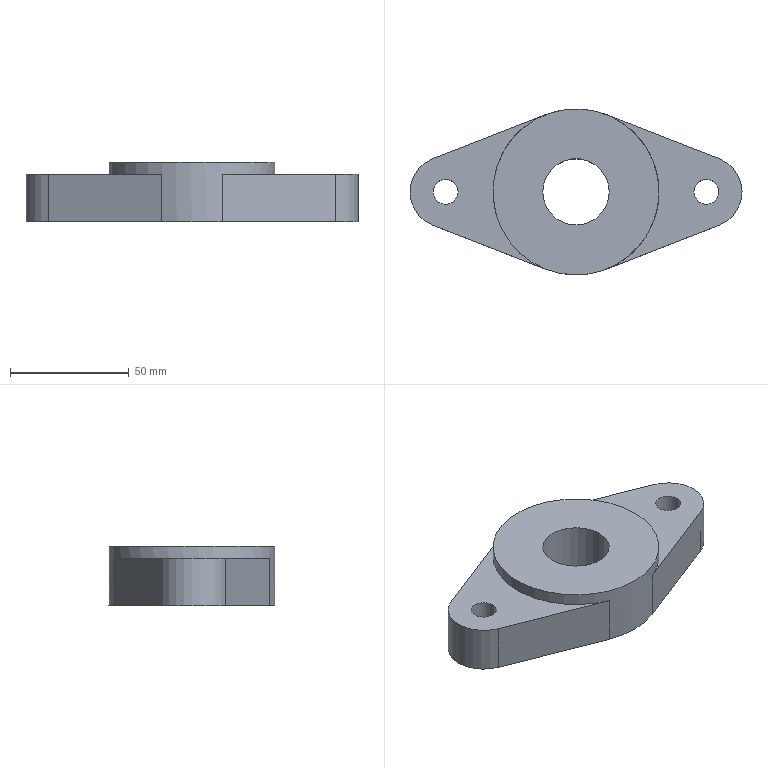Component | NX | FIXED_PLATE | 1 solid | 14 faces | box 140 x 70 x 25 mm | volume 131878 mm3 | plane 8 | cylinder 6 | commonest cylinder face diameters 30 x2 10.5 x2 70 x1 28 x1
STEP:
#1=CARTESIAN_POINT('',(0.,0.,0.));
#2=DIRECTION('',(0.,0.,1.));
#3=DIRECTION('',(1.,0.,0.));
#4=AXIS2_PLACEMENT_3D('',#1,#2,#3);
#5=CARTESIAN_POINT('',(-12.727,-32.604,162.5));
#6=VERTEX_POINT('',#5);
#7=CARTESIAN_POINT('',(-12.727,32.604,162.5));
#8=VERTEX_POINT('',#7);
#9=CARTESIAN_POINT('',(-0.,-0.,162.5));
#10=DIRECTION('',(0.,0.,-1.));
#11=DIRECTION('',(1.,0.,0.));
#12=AXIS2_PLACEMENT_3D('',#9,#10,#11);
#13=CIRCLE('',#12,35.);
#14=CARTESIAN_POINT('',(-55.,-0.,162.5));
#15=DIRECTION('',(0.,0.,1.));
#16=DIRECTION('',(1.,0.,0.));
#17=AXIS2_PLACEMENT_3D('',#14,#15,#16);
#18=PLANE('',#17);
#19=CARTESIAN_POINT('',(90.,0.));
#20=CARTESIAN_POINT('',(90.,-60.622));
#21=CARTESIAN_POINT('',(37.5,-30.311));
#22=CARTESIAN_POINT('',(-15.,-0.));
#23=CARTESIAN_POINT('',(37.5,30.311));
#24=CARTESIAN_POINT('',(90.,60.622));
#25=CARTESIAN_POINT('',(90.,0.));
#26=(BOUNDED_CURVE()B_SPLINE_CURVE(2,(#19,#20,#21,#22,#23,#24,#25),.UNSPECIFIED.,.T.,.F.)B_SPLINE_CURVE_WITH_KNOTS((1,2,2,2,2,1),(-2.094,0.,2.094,4.189,6.283,8.378),.UNSPECIFIED.)CURVE()GEOMETRIC_REPRESENTATION_ITEM()RATIONAL_B_SPLINE_CURVE((1.,0.5,1.,0.5,1.,0.5,1.))REPRESENTATION_ITEM(''));
#27=(GEOMETRIC_REPRESENTATION_CONTEXT(2)PARAMETRIC_REPRESENTATION_CONTEXT()REPRESENTATION_CONTEXT('',''));
#28=DEFINITIONAL_REPRESENTATION('',(#26),#27);
#29=PCURVE('',#18,#28);
#30=CARTESIAN_POINT('',(-0.,-0.,162.5));
#31=DIRECTION('',(0.,0.,-1.));
#32=DIRECTION('',(-1.,0.,0.));
#33=AXIS2_PLACEMENT_3D('',#30,#31,#32);
#34=CYLINDRICAL_SURFACE('',#33,35.);
#35=CARTESIAN_POINT('',(3.142,0.));
#36=DIRECTION('',(1.,0.));
#37=VECTOR('',#36,1.);
#38=LINE('',#35,#37);
#39=(GEOMETRIC_REPRESENTATION_CONTEXT(2)PARAMETRIC_REPRESENTATION_CONTEXT()REPRESENTATION_CONTEXT('',''));
#40=DEFINITIONAL_REPRESENTATION('',(#38),#39);
#41=PCURVE('',#34,#40);
#42=SURFACE_CURVE('',#13,(#29,#41),.PCURVE_S1.);
#43=EDGE_CURVE('',#6,#8,#42,.T.);
#44=ORIENTED_EDGE('',*,*,#43,.T.);
#45=CARTESIAN_POINT('',(-60.455,13.973,162.5));
#46=VERTEX_POINT('',#45);
#47=CARTESIAN_POINT('',(-12.727,32.604,162.5));
#48=DIRECTION('',(-0.9315,-0.3636,0.));
#49=VECTOR('',#48,1.);
#50=LINE('',#47,#49);
#51=CARTESIAN_POINT('',(42.273,32.604));
#52=DIRECTION('',(-0.9315,-0.3636));
#53=VECTOR('',#52,1.);
#54=LINE('',#51,#53);
#55=(GEOMETRIC_REPRESENTATION_CONTEXT(2)PARAMETRIC_REPRESENTATION_CONTEXT()REPRESENTATION_CONTEXT('',''));
#56=DEFINITIONAL_REPRESENTATION('',(#54),#55);
#57=PCURVE('',#18,#56);
#58=CARTESIAN_POINT('',(-12.727,32.604,162.5));
#59=DIRECTION('',(0.3636,-0.9315,0.));
#60=DIRECTION('',(0.9315,0.3636,0.));
#61=AXIS2_PLACEMENT_3D('',#58,#59,#60);
#62=PLANE('',#61);
#63=CARTESIAN_POINT('',(0.,0.));
#64=DIRECTION('',(-1.,0.));
#65=VECTOR('',#64,1.);
#66=LINE('',#63,#65);
#67=(GEOMETRIC_REPRESENTATION_CONTEXT(2)PARAMETRIC_REPRESENTATION_CONTEXT()REPRESENTATION_CONTEXT('',''));
#68=DEFINITIONAL_REPRESENTATION('',(#66),#67);
#69=PCURVE('',#62,#68);
#70=SURFACE_CURVE('',#50,(#57,#69),.PCURVE_S1.);
#71=EDGE_CURVE('',#8,#46,#70,.T.);
#72=ORIENTED_EDGE('',*,*,#71,.T.);
#73=CARTESIAN_POINT('',(-60.455,-13.973,162.5));
#74=VERTEX_POINT('',#73);
#75=CARTESIAN_POINT('',(-55.,-0.,162.5));
#76=DIRECTION('',(0.,0.,1.));
#77=DIRECTION('',(1.,0.,0.));
#78=AXIS2_PLACEMENT_3D('',#75,#76,#77);
#79=CIRCLE('',#78,15.);
#80=CARTESIAN_POINT('',(0.,0.));
#81=DIRECTION('',(1.,0.));
#82=AXIS2_PLACEMENT_2D('',#80,#81);
#83=CIRCLE('',#82,15.);
#84=(GEOMETRIC_REPRESENTATION_CONTEXT(2)PARAMETRIC_REPRESENTATION_CONTEXT()REPRESENTATION_CONTEXT('',''));
#85=DEFINITIONAL_REPRESENTATION('',(#83),#84);
#86=PCURVE('',#18,#85);
#87=CARTESIAN_POINT('',(-55.,-0.,162.5));
#88=DIRECTION('',(0.,0.,-1.));
#89=DIRECTION('',(-1.,0.,0.));
#90=AXIS2_PLACEMENT_3D('',#87,#88,#89);
#91=CYLINDRICAL_SURFACE('',#90,15.);
#92=CARTESIAN_POINT('',(3.142,0.));
#93=DIRECTION('',(-1.,0.));
#94=VECTOR('',#93,1.);
#95=LINE('',#92,#94);
#96=(GEOMETRIC_REPRESENTATION_CONTEXT(2)PARAMETRIC_REPRESENTATION_CONTEXT()REPRESENTATION_CONTEXT('',''));
#97=DEFINITIONAL_REPRESENTATION('',(#95),#96);
#98=PCURVE('',#91,#97);
#99=SURFACE_CURVE('',#79,(#86,#98),.PCURVE_S1.);
#100=EDGE_CURVE('',#46,#74,#99,.T.);
#101=ORIENTED_EDGE('',*,*,#100,.T.);
#102=CARTESIAN_POINT('',(-60.455,-13.973,162.5));
#103=DIRECTION('',(0.9315,-0.3636,0.));
#104=VECTOR('',#103,1.);
#105=LINE('',#102,#104);
#106=CARTESIAN_POINT('',(-5.455,-13.973));
#107=DIRECTION('',(0.9315,-0.3636));
#108=VECTOR('',#107,1.);
#109=LINE('',#106,#108);
#110=(GEOMETRIC_REPRESENTATION_CONTEXT(2)PARAMETRIC_REPRESENTATION_CONTEXT()REPRESENTATION_CONTEXT('',''));
#111=DEFINITIONAL_REPRESENTATION('',(#109),#110);
#112=PCURVE('',#18,#111);
#113=CARTESIAN_POINT('',(-60.455,-13.973,162.5));
#114=DIRECTION('',(0.3636,0.9315,0.));
#115=DIRECTION('',(-0.9315,0.3636,0.));
#116=AXIS2_PLACEMENT_3D('',#113,#114,#115);
#117=PLANE('',#116);
#118=CARTESIAN_POINT('',(0.,0.));
#119=DIRECTION('',(-1.,0.));
#120=VECTOR('',#119,1.);
#121=LINE('',#118,#120);
#122=(GEOMETRIC_REPRESENTATION_CONTEXT(2)PARAMETRIC_REPRESENTATION_CONTEXT()REPRESENTATION_CONTEXT('',''));
#123=DEFINITIONAL_REPRESENTATION('',(#121),#122);
#124=PCURVE('',#117,#123);
#125=SURFACE_CURVE('',#105,(#112,#124),.PCURVE_S1.);
#126=EDGE_CURVE('',#74,#6,#125,.T.);
#127=ORIENTED_EDGE('',*,*,#126,.T.);
#128=EDGE_LOOP('',(#44,#72,#101,#127));
#129=FACE_BOUND('',#128,.T.);
#130=CARTESIAN_POINT('',(-49.75,-0.,162.5));
#131=VERTEX_POINT('',#130);
#132=CARTESIAN_POINT('',(-55.,-0.,162.5));
#133=DIRECTION('',(0.,0.,1.));
#134=DIRECTION('',(1.,0.,0.));
#135=AXIS2_PLACEMENT_3D('',#132,#133,#134);
#136=CIRCLE('',#135,5.25);
#137=CARTESIAN_POINT('',(0.,0.));
#138=DIRECTION('',(1.,0.));
#139=AXIS2_PLACEMENT_2D('',#137,#138);
#140=CIRCLE('',#139,5.25);
#141=(GEOMETRIC_REPRESENTATION_CONTEXT(2)PARAMETRIC_REPRESENTATION_CONTEXT()REPRESENTATION_CONTEXT('',''));
#142=DEFINITIONAL_REPRESENTATION('',(#140),#141);
#143=PCURVE('',#18,#142);
#144=CARTESIAN_POINT('',(-55.,-0.,162.5));
#145=DIRECTION('',(0.,0.,-1.));
#146=DIRECTION('',(-1.,0.,0.));
#147=AXIS2_PLACEMENT_3D('',#144,#145,#146);
#148=CYLINDRICAL_SURFACE('',#147,5.25);
#149=CARTESIAN_POINT('',(9.425,0.));
#150=DIRECTION('',(-1.,0.));
#151=VECTOR('',#150,1.);
#152=LINE('',#149,#151);
#153=(GEOMETRIC_REPRESENTATION_CONTEXT(2)PARAMETRIC_REPRESENTATION_CONTEXT()REPRESENTATION_CONTEXT('',''));
#154=DEFINITIONAL_REPRESENTATION('',(#152),#153);
#155=PCURVE('',#148,#154);
#156=SURFACE_CURVE('',#136,(#143,#155),.PCURVE_S1.);
#157=EDGE_CURVE('',#131,#131,#156,.T.);
#158=ORIENTED_EDGE('',*,*,#157,.F.);
#159=EDGE_LOOP('',(#158));
#160=FACE_BOUND('',#159,.T.);
#161=ADVANCED_FACE('',(#129,#160),#18,.T.);
#162=CARTESIAN_POINT('',(-60.455,13.973,142.5));
#163=VERTEX_POINT('',#162);
#164=CARTESIAN_POINT('',(-60.455,-13.973,142.5));
#165=VERTEX_POINT('',#164);
#166=CARTESIAN_POINT('',(-55.,-0.,142.5));
#167=DIRECTION('',(0.,0.,1.));
#168=DIRECTION('',(1.,0.,0.));
#169=AXIS2_PLACEMENT_3D('',#166,#167,#168);
#170=CIRCLE('',#169,15.);
#171=CARTESIAN_POINT('',(3.142,20.));
#172=DIRECTION('',(-1.,0.));
#173=VECTOR('',#172,1.);
#174=LINE('',#171,#173);
#175=(GEOMETRIC_REPRESENTATION_CONTEXT(2)PARAMETRIC_REPRESENTATION_CONTEXT()REPRESENTATION_CONTEXT('',''));
#176=DEFINITIONAL_REPRESENTATION('',(#174),#175);
#177=PCURVE('',#91,#176);
#178=CARTESIAN_POINT('',(-55.,-0.,142.5));
#179=DIRECTION('',(0.,0.,1.));
#180=DIRECTION('',(1.,0.,0.));
#181=AXIS2_PLACEMENT_3D('',#178,#179,#180);
#182=PLANE('',#181);
#183=CARTESIAN_POINT('',(0.,0.));
#184=DIRECTION('',(1.,0.));
#185=AXIS2_PLACEMENT_2D('',#183,#184);
#186=CIRCLE('',#185,15.);
#187=(GEOMETRIC_REPRESENTATION_CONTEXT(2)PARAMETRIC_REPRESENTATION_CONTEXT()REPRESENTATION_CONTEXT('',''));
#188=DEFINITIONAL_REPRESENTATION('',(#186),#187);
#189=PCURVE('',#182,#188);
#190=SURFACE_CURVE('',#170,(#177,#189),.PCURVE_S1.);
#191=EDGE_CURVE('',#163,#165,#190,.T.);
#192=ORIENTED_EDGE('',*,*,#191,.T.);
#193=CARTESIAN_POINT('',(-60.455,-13.973,162.5));
#194=DIRECTION('',(0.,0.,-1.));
#195=VECTOR('',#194,1.);
#196=LINE('',#193,#195);
#197=CARTESIAN_POINT('',(-1.199,0.));
#198=DIRECTION('',(0.,1.));
#199=VECTOR('',#198,1.);
#200=LINE('',#197,#199);
#201=(GEOMETRIC_REPRESENTATION_CONTEXT(2)PARAMETRIC_REPRESENTATION_CONTEXT()REPRESENTATION_CONTEXT('',''));
#202=DEFINITIONAL_REPRESENTATION('',(#200),#201);
#203=PCURVE('',#91,#202);
#204=CARTESIAN_POINT('',(0.,0.));
#205=DIRECTION('',(0.,-1.));
#206=VECTOR('',#205,1.);
#207=LINE('',#204,#206);
#208=(GEOMETRIC_REPRESENTATION_CONTEXT(2)PARAMETRIC_REPRESENTATION_CONTEXT()REPRESENTATION_CONTEXT('',''));
#209=DEFINITIONAL_REPRESENTATION('',(#207),#208);
#210=PCURVE('',#117,#209);
#211=SURFACE_CURVE('',#196,(#203,#210),.PCURVE_S1.);
#212=EDGE_CURVE('',#74,#165,#211,.T.);
#213=ORIENTED_EDGE('',*,*,#212,.F.);
#214=ORIENTED_EDGE('',*,*,#100,.F.);
#215=CARTESIAN_POINT('',(-60.455,13.973,162.5));
#216=DIRECTION('',(0.,0.,-1.));
#217=VECTOR('',#216,1.);
#218=LINE('',#215,#217);
#219=CARTESIAN_POINT('',(1.199,0.));
#220=DIRECTION('',(0.,1.));
#221=VECTOR('',#220,1.);
#222=LINE('',#219,#221);
#223=(GEOMETRIC_REPRESENTATION_CONTEXT(2)PARAMETRIC_REPRESENTATION_CONTEXT()REPRESENTATION_CONTEXT('',''));
#224=DEFINITIONAL_REPRESENTATION('',(#222),#223);
#225=PCURVE('',#91,#224);
#226=CARTESIAN_POINT('',(-51.235,0.));
#227=DIRECTION('',(0.,-1.));
#228=VECTOR('',#227,1.);
#229=LINE('',#226,#228);
#230=(GEOMETRIC_REPRESENTATION_CONTEXT(2)PARAMETRIC_REPRESENTATION_CONTEXT()REPRESENTATION_CONTEXT('',''));
#231=DEFINITIONAL_REPRESENTATION('',(#229),#230);
#232=PCURVE('',#62,#231);
#233=SURFACE_CURVE('',#218,(#225,#232),.PCURVE_S1.);
#234=EDGE_CURVE('',#46,#163,#233,.T.);
#235=ORIENTED_EDGE('',*,*,#234,.T.);
#236=EDGE_LOOP('',(#192,#213,#214,#235));
#237=FACE_BOUND('',#236,.T.);
#238=ADVANCED_FACE('',(#237),#91,.T.);
#239=CARTESIAN_POINT('',(-12.727,-32.604,142.5));
#240=VERTEX_POINT('',#239);
#241=CARTESIAN_POINT('',(-60.455,-13.973,142.5));
#242=DIRECTION('',(0.9315,-0.3636,0.));
#243=VECTOR('',#242,1.);
#244=LINE('',#241,#243);
#245=CARTESIAN_POINT('',(0.,-20.));
#246=DIRECTION('',(-1.,0.));
#247=VECTOR('',#246,1.);
#248=LINE('',#245,#247);
#249=(GEOMETRIC_REPRESENTATION_CONTEXT(2)PARAMETRIC_REPRESENTATION_CONTEXT()REPRESENTATION_CONTEXT('',''));
#250=DEFINITIONAL_REPRESENTATION('',(#248),#249);
#251=PCURVE('',#117,#250);
#252=CARTESIAN_POINT('',(-5.455,-13.973));
#253=DIRECTION('',(0.9315,-0.3636));
#254=VECTOR('',#253,1.);
#255=LINE('',#252,#254);
#256=(GEOMETRIC_REPRESENTATION_CONTEXT(2)PARAMETRIC_REPRESENTATION_CONTEXT()REPRESENTATION_CONTEXT('',''));
#257=DEFINITIONAL_REPRESENTATION('',(#255),#256);
#258=PCURVE('',#182,#257);
#259=SURFACE_CURVE('',#244,(#251,#258),.PCURVE_S1.);
#260=EDGE_CURVE('',#165,#240,#259,.T.);
#261=ORIENTED_EDGE('',*,*,#260,.T.);
#262=CARTESIAN_POINT('',(-12.727,-32.604,162.5));
#263=DIRECTION('',(0.,0.,-1.));
#264=VECTOR('',#263,1.);
#265=LINE('',#262,#264);
#266=CARTESIAN_POINT('',(-51.235,0.));
#267=DIRECTION('',(0.,-1.));
#268=VECTOR('',#267,1.);
#269=LINE('',#266,#268);
#270=(GEOMETRIC_REPRESENTATION_CONTEXT(2)PARAMETRIC_REPRESENTATION_CONTEXT()REPRESENTATION_CONTEXT('',''));
#271=DEFINITIONAL_REPRESENTATION('',(#269),#270);
#272=PCURVE('',#117,#271);
#273=CARTESIAN_POINT('',(11.368,0.));
#274=DIRECTION('',(0.,1.));
#275=VECTOR('',#274,1.);
#276=LINE('',#273,#275);
#277=(GEOMETRIC_REPRESENTATION_CONTEXT(2)PARAMETRIC_REPRESENTATION_CONTEXT()REPRESENTATION_CONTEXT('',''));
#278=DEFINITIONAL_REPRESENTATION('',(#276),#277);
#279=PCURVE('',#34,#278);
#280=SURFACE_CURVE('',#265,(#272,#279),.PCURVE_S1.);
#281=EDGE_CURVE('',#6,#240,#280,.T.);
#282=ORIENTED_EDGE('',*,*,#281,.F.);
#283=ORIENTED_EDGE('',*,*,#126,.F.);
#284=ORIENTED_EDGE('',*,*,#212,.T.);
#285=EDGE_LOOP('',(#261,#282,#283,#284));
#286=FACE_BOUND('',#285,.T.);
#287=ADVANCED_FACE('',(#286),#117,.F.);
#288=CARTESIAN_POINT('',(12.727,-32.604,142.5));
#289=VERTEX_POINT('',#288);
#290=CARTESIAN_POINT('',(60.455,-13.973,142.5));
#291=VERTEX_POINT('',#290);
#292=CARTESIAN_POINT('',(12.727,-32.604,142.5));
#293=DIRECTION('',(0.9315,0.3636,0.));
#294=VECTOR('',#293,1.);
#295=LINE('',#292,#294);
#296=CARTESIAN_POINT('',(12.727,-32.604,162.5));
#297=DIRECTION('',(-0.3636,0.9315,0.));
#298=DIRECTION('',(-0.9315,-0.3636,0.));
#299=AXIS2_PLACEMENT_3D('',#296,#297,#298);
#300=PLANE('',#299);
#301=CARTESIAN_POINT('',(0.,-20.));
#302=DIRECTION('',(-1.,0.));
#303=VECTOR('',#302,1.);
#304=LINE('',#301,#303);
#305=(GEOMETRIC_REPRESENTATION_CONTEXT(2)PARAMETRIC_REPRESENTATION_CONTEXT()REPRESENTATION_CONTEXT('',''));
#306=DEFINITIONAL_REPRESENTATION('',(#304),#305);
#307=PCURVE('',#300,#306);
#308=CARTESIAN_POINT('',(67.727,-32.604));
#309=DIRECTION('',(0.9315,0.3636));
#310=VECTOR('',#309,1.);
#311=LINE('',#308,#310);
#312=(GEOMETRIC_REPRESENTATION_CONTEXT(2)PARAMETRIC_REPRESENTATION_CONTEXT()REPRESENTATION_CONTEXT('',''));
#313=DEFINITIONAL_REPRESENTATION('',(#311),#312);
#314=PCURVE('',#182,#313);
#315=SURFACE_CURVE('',#295,(#307,#314),.PCURVE_S1.);
#316=EDGE_CURVE('',#289,#291,#315,.T.);
#317=ORIENTED_EDGE('',*,*,#316,.T.);
#318=CARTESIAN_POINT('',(60.455,-13.973,162.5));
#319=VERTEX_POINT('',#318);
#320=CARTESIAN_POINT('',(60.455,-13.973,162.5));
#321=DIRECTION('',(0.,0.,-1.));
#322=VECTOR('',#321,1.);
#323=LINE('',#320,#322);
#324=CARTESIAN_POINT('',(-51.235,0.));
#325=DIRECTION('',(0.,-1.));
#326=VECTOR('',#325,1.);
#327=LINE('',#324,#326);
#328=(GEOMETRIC_REPRESENTATION_CONTEXT(2)PARAMETRIC_REPRESENTATION_CONTEXT()REPRESENTATION_CONTEXT('',''));
#329=DEFINITIONAL_REPRESENTATION('',(#327),#328);
#330=PCURVE('',#300,#329);
#331=CARTESIAN_POINT('',(55.,-0.,162.5));
#332=DIRECTION('',(0.,0.,-1.));
#333=DIRECTION('',(-1.,0.,0.));
#334=AXIS2_PLACEMENT_3D('',#331,#332,#333);
#335=CYLINDRICAL_SURFACE('',#334,15.);
#336=CARTESIAN_POINT('',(4.34,0.));
#337=DIRECTION('',(0.,1.));
#338=VECTOR('',#337,1.);
#339=LINE('',#336,#338);
#340=(GEOMETRIC_REPRESENTATION_CONTEXT(2)PARAMETRIC_REPRESENTATION_CONTEXT()REPRESENTATION_CONTEXT('',''));
#341=DEFINITIONAL_REPRESENTATION('',(#339),#340);
#342=PCURVE('',#335,#341);
#343=SURFACE_CURVE('',#323,(#330,#342),.PCURVE_S1.);
#344=EDGE_CURVE('',#319,#291,#343,.T.);
#345=ORIENTED_EDGE('',*,*,#344,.F.);
#346=CARTESIAN_POINT('',(12.727,-32.604,162.5));
#347=VERTEX_POINT('',#346);
#348=CARTESIAN_POINT('',(12.727,-32.604,162.5));
#349=DIRECTION('',(0.9315,0.3636,0.));
#350=VECTOR('',#349,1.);
#351=LINE('',#348,#350);
#352=CARTESIAN_POINT('',(0.,0.));
#353=DIRECTION('',(-1.,0.));
#354=VECTOR('',#353,1.);
#355=LINE('',#352,#354);
#356=(GEOMETRIC_REPRESENTATION_CONTEXT(2)PARAMETRIC_REPRESENTATION_CONTEXT()REPRESENTATION_CONTEXT('',''));
#357=DEFINITIONAL_REPRESENTATION('',(#355),#356);
#358=PCURVE('',#300,#357);
#359=CARTESIAN_POINT('',(-55.,-0.,162.5));
#360=DIRECTION('',(0.,0.,1.));
#361=DIRECTION('',(1.,0.,0.));
#362=AXIS2_PLACEMENT_3D('',#359,#360,#361);
#363=PLANE('',#362);
#364=CARTESIAN_POINT('',(67.727,-32.604));
#365=DIRECTION('',(0.9315,0.3636));
#366=VECTOR('',#365,1.);
#367=LINE('',#364,#366);
#368=(GEOMETRIC_REPRESENTATION_CONTEXT(2)PARAMETRIC_REPRESENTATION_CONTEXT()REPRESENTATION_CONTEXT('',''));
#369=DEFINITIONAL_REPRESENTATION('',(#367),#368);
#370=PCURVE('',#363,#369);
#371=SURFACE_CURVE('',#351,(#358,#370),.PCURVE_S1.);
#372=EDGE_CURVE('',#347,#319,#371,.T.);
#373=ORIENTED_EDGE('',*,*,#372,.F.);
#374=CARTESIAN_POINT('',(12.727,-32.604,162.5));
#375=DIRECTION('',(0.,0.,-1.));
#376=VECTOR('',#375,1.);
#377=LINE('',#374,#376);
#378=CARTESIAN_POINT('',(0.,0.));
#379=DIRECTION('',(0.,-1.));
#380=VECTOR('',#379,1.);
#381=LINE('',#378,#380);
#382=(GEOMETRIC_REPRESENTATION_CONTEXT(2)PARAMETRIC_REPRESENTATION_CONTEXT()REPRESENTATION_CONTEXT('',''));
#383=DEFINITIONAL_REPRESENTATION('',(#381),#382);
#384=PCURVE('',#300,#383);
#385=CARTESIAN_POINT('',(10.623,0.));
#386=DIRECTION('',(0.,1.));
#387=VECTOR('',#386,1.);
#388=LINE('',#385,#387);
#389=(GEOMETRIC_REPRESENTATION_CONTEXT(2)PARAMETRIC_REPRESENTATION_CONTEXT()REPRESENTATION_CONTEXT('',''));
#390=DEFINITIONAL_REPRESENTATION('',(#388),#389);
#391=PCURVE('',#34,#390);
#392=SURFACE_CURVE('',#377,(#384,#391),.PCURVE_S1.);
#393=EDGE_CURVE('',#347,#289,#392,.T.);
#394=ORIENTED_EDGE('',*,*,#393,.T.);
#395=EDGE_LOOP('',(#317,#345,#373,#394));
#396=FACE_BOUND('',#395,.T.);
#397=ADVANCED_FACE('',(#396),#300,.F.);
#398=CARTESIAN_POINT('',(60.455,13.973,142.5));
#399=VERTEX_POINT('',#398);
#400=CARTESIAN_POINT('',(55.,-0.,142.5));
#401=DIRECTION('',(0.,0.,1.));
#402=DIRECTION('',(-1.,0.,0.));
#403=AXIS2_PLACEMENT_3D('',#400,#401,#402);
#404=CIRCLE('',#403,15.);
#405=CARTESIAN_POINT('',(6.283,20.));
#406=DIRECTION('',(-1.,0.));
#407=VECTOR('',#406,1.);
#408=LINE('',#405,#407);
#409=(GEOMETRIC_REPRESENTATION_CONTEXT(2)PARAMETRIC_REPRESENTATION_CONTEXT()REPRESENTATION_CONTEXT('',''));
#410=DEFINITIONAL_REPRESENTATION('',(#408),#409);
#411=PCURVE('',#335,#410);
#412=CARTESIAN_POINT('',(110.,0.));
#413=DIRECTION('',(-1.,0.));
#414=AXIS2_PLACEMENT_2D('',#412,#413);
#415=CIRCLE('',#414,15.);
#416=(GEOMETRIC_REPRESENTATION_CONTEXT(2)PARAMETRIC_REPRESENTATION_CONTEXT()REPRESENTATION_CONTEXT('',''));
#417=DEFINITIONAL_REPRESENTATION('',(#415),#416);
#418=PCURVE('',#182,#417);
#419=SURFACE_CURVE('',#404,(#411,#418),.PCURVE_S1.);
#420=EDGE_CURVE('',#291,#399,#419,.T.);
#421=ORIENTED_EDGE('',*,*,#420,.T.);
#422=CARTESIAN_POINT('',(60.455,13.973,162.5));
#423=VERTEX_POINT('',#422);
#424=CARTESIAN_POINT('',(60.455,13.973,162.5));
#425=DIRECTION('',(0.,0.,-1.));
#426=VECTOR('',#425,1.);
#427=LINE('',#424,#426);
#428=CARTESIAN_POINT('',(1.943,0.));
#429=DIRECTION('',(0.,1.));
#430=VECTOR('',#429,1.);
#431=LINE('',#428,#430);
#432=(GEOMETRIC_REPRESENTATION_CONTEXT(2)PARAMETRIC_REPRESENTATION_CONTEXT()REPRESENTATION_CONTEXT('',''));
#433=DEFINITIONAL_REPRESENTATION('',(#431),#432);
#434=PCURVE('',#335,#433);
#435=CARTESIAN_POINT('',(60.455,13.973,162.5));
#436=DIRECTION('',(-0.3636,-0.9315,0.));
#437=DIRECTION('',(0.9315,-0.3636,0.));
#438=AXIS2_PLACEMENT_3D('',#435,#436,#437);
#439=PLANE('',#438);
#440=CARTESIAN_POINT('',(0.,0.));
#441=DIRECTION('',(0.,-1.));
#442=VECTOR('',#441,1.);
#443=LINE('',#440,#442);
#444=(GEOMETRIC_REPRESENTATION_CONTEXT(2)PARAMETRIC_REPRESENTATION_CONTEXT()REPRESENTATION_CONTEXT('',''));
#445=DEFINITIONAL_REPRESENTATION('',(#443),#444);
#446=PCURVE('',#439,#445);
#447=SURFACE_CURVE('',#427,(#434,#446),.PCURVE_S1.);
#448=EDGE_CURVE('',#423,#399,#447,.T.);
#449=ORIENTED_EDGE('',*,*,#448,.F.);
#450=CARTESIAN_POINT('',(55.,-0.,162.5));
#451=DIRECTION('',(0.,0.,1.));
#452=DIRECTION('',(-1.,0.,0.));
#453=AXIS2_PLACEMENT_3D('',#450,#451,#452);
#454=CIRCLE('',#453,15.);
#455=CARTESIAN_POINT('',(6.283,0.));
#456=DIRECTION('',(-1.,0.));
#457=VECTOR('',#456,1.);
#458=LINE('',#455,#457);
#459=(GEOMETRIC_REPRESENTATION_CONTEXT(2)PARAMETRIC_REPRESENTATION_CONTEXT()REPRESENTATION_CONTEXT('',''));
#460=DEFINITIONAL_REPRESENTATION('',(#458),#459);
#461=PCURVE('',#335,#460);
#462=CARTESIAN_POINT('',(110.,0.));
#463=DIRECTION('',(-1.,0.));
#464=AXIS2_PLACEMENT_2D('',#462,#463);
#465=CIRCLE('',#464,15.);
#466=(GEOMETRIC_REPRESENTATION_CONTEXT(2)PARAMETRIC_REPRESENTATION_CONTEXT()REPRESENTATION_CONTEXT('',''));
#467=DEFINITIONAL_REPRESENTATION('',(#465),#466);
#468=PCURVE('',#363,#467);
#469=SURFACE_CURVE('',#454,(#461,#468),.PCURVE_S1.);
#470=EDGE_CURVE('',#319,#423,#469,.T.);
#471=ORIENTED_EDGE('',*,*,#470,.F.);
#472=ORIENTED_EDGE('',*,*,#344,.T.);
#473=EDGE_LOOP('',(#421,#449,#471,#472));
#474=FACE_BOUND('',#473,.T.);
#475=ADVANCED_FACE('',(#474),#335,.T.);
#476=CARTESIAN_POINT('',(12.727,32.604,142.5));
#477=VERTEX_POINT('',#476);
#478=CARTESIAN_POINT('',(60.455,13.973,142.5));
#479=DIRECTION('',(-0.9315,0.3636,0.));
#480=VECTOR('',#479,1.);
#481=LINE('',#478,#480);
#482=CARTESIAN_POINT('',(0.,-20.));
#483=DIRECTION('',(-1.,0.));
#484=VECTOR('',#483,1.);
#485=LINE('',#482,#484);
#486=(GEOMETRIC_REPRESENTATION_CONTEXT(2)PARAMETRIC_REPRESENTATION_CONTEXT()REPRESENTATION_CONTEXT('',''));
#487=DEFINITIONAL_REPRESENTATION('',(#485),#486);
#488=PCURVE('',#439,#487);
#489=CARTESIAN_POINT('',(115.455,13.973));
#490=DIRECTION('',(-0.9315,0.3636));
#491=VECTOR('',#490,1.);
#492=LINE('',#489,#491);
#493=(GEOMETRIC_REPRESENTATION_CONTEXT(2)PARAMETRIC_REPRESENTATION_CONTEXT()REPRESENTATION_CONTEXT('',''));
#494=DEFINITIONAL_REPRESENTATION('',(#492),#493);
#495=PCURVE('',#182,#494);
#496=SURFACE_CURVE('',#481,(#488,#495),.PCURVE_S1.);
#497=EDGE_CURVE('',#399,#477,#496,.T.);
#498=ORIENTED_EDGE('',*,*,#497,.T.);
#499=CARTESIAN_POINT('',(12.727,32.604,162.5));
#500=VERTEX_POINT('',#499);
#501=CARTESIAN_POINT('',(12.727,32.604,162.5));
#502=DIRECTION('',(0.,0.,-1.));
#503=VECTOR('',#502,1.);
#504=LINE('',#501,#503);
#505=CARTESIAN_POINT('',(-51.235,0.));
#506=DIRECTION('',(0.,-1.));
#507=VECTOR('',#506,1.);
#508=LINE('',#505,#507);
#509=(GEOMETRIC_REPRESENTATION_CONTEXT(2)PARAMETRIC_REPRESENTATION_CONTEXT()REPRESENTATION_CONTEXT('',''));
#510=DEFINITIONAL_REPRESENTATION('',(#508),#509);
#511=PCURVE('',#439,#510);
#512=CARTESIAN_POINT('',(8.226,0.));
#513=DIRECTION('',(0.,1.));
#514=VECTOR('',#513,1.);
#515=LINE('',#512,#514);
#516=(GEOMETRIC_REPRESENTATION_CONTEXT(2)PARAMETRIC_REPRESENTATION_CONTEXT()REPRESENTATION_CONTEXT('',''));
#517=DEFINITIONAL_REPRESENTATION('',(#515),#516);
#518=PCURVE('',#34,#517);
#519=SURFACE_CURVE('',#504,(#511,#518),.PCURVE_S1.);
#520=EDGE_CURVE('',#500,#477,#519,.T.);
#521=ORIENTED_EDGE('',*,*,#520,.F.);
#522=CARTESIAN_POINT('',(60.455,13.973,162.5));
#523=DIRECTION('',(-0.9315,0.3636,0.));
#524=VECTOR('',#523,1.);
#525=LINE('',#522,#524);
#526=CARTESIAN_POINT('',(0.,0.));
#527=DIRECTION('',(-1.,0.));
#528=VECTOR('',#527,1.);
#529=LINE('',#526,#528);
#530=(GEOMETRIC_REPRESENTATION_CONTEXT(2)PARAMETRIC_REPRESENTATION_CONTEXT()REPRESENTATION_CONTEXT('',''));
#531=DEFINITIONAL_REPRESENTATION('',(#529),#530);
#532=PCURVE('',#439,#531);
#533=CARTESIAN_POINT('',(115.455,13.973));
#534=DIRECTION('',(-0.9315,0.3636));
#535=VECTOR('',#534,1.);
#536=LINE('',#533,#535);
#537=(GEOMETRIC_REPRESENTATION_CONTEXT(2)PARAMETRIC_REPRESENTATION_CONTEXT()REPRESENTATION_CONTEXT('',''));
#538=DEFINITIONAL_REPRESENTATION('',(#536),#537);
#539=PCURVE('',#363,#538);
#540=SURFACE_CURVE('',#525,(#532,#539),.PCURVE_S1.);
#541=EDGE_CURVE('',#423,#500,#540,.T.);
#542=ORIENTED_EDGE('',*,*,#541,.F.);
#543=ORIENTED_EDGE('',*,*,#448,.T.);
#544=EDGE_LOOP('',(#498,#521,#542,#543));
#545=FACE_BOUND('',#544,.T.);
#546=ADVANCED_FACE('',(#545),#439,.F.);
#547=CARTESIAN_POINT('',(-12.727,32.604,142.5));
#548=VERTEX_POINT('',#547);
#549=CARTESIAN_POINT('',(-0.,-0.,142.5));
#550=DIRECTION('',(0.,0.,1.));
#551=DIRECTION('',(1.,0.,0.));
#552=AXIS2_PLACEMENT_3D('',#549,#550,#551);
#553=CIRCLE('',#552,35.);
#554=CARTESIAN_POINT('',(9.425,20.));
#555=DIRECTION('',(-1.,0.));
#556=VECTOR('',#555,1.);
#557=LINE('',#554,#556);
#558=(GEOMETRIC_REPRESENTATION_CONTEXT(2)PARAMETRIC_REPRESENTATION_CONTEXT()REPRESENTATION_CONTEXT('',''));
#559=DEFINITIONAL_REPRESENTATION('',(#557),#558);
#560=PCURVE('',#34,#559);
#561=CARTESIAN_POINT('',(55.,0.));
#562=DIRECTION('',(1.,0.));
#563=AXIS2_PLACEMENT_2D('',#561,#562);
#564=CIRCLE('',#563,35.);
#565=(GEOMETRIC_REPRESENTATION_CONTEXT(2)PARAMETRIC_REPRESENTATION_CONTEXT()REPRESENTATION_CONTEXT('',''));
#566=DEFINITIONAL_REPRESENTATION('',(#564),#565);
#567=PCURVE('',#182,#566);
#568=SURFACE_CURVE('',#553,(#560,#567),.PCURVE_S1.);
#569=EDGE_CURVE('',#477,#548,#568,.T.);
#570=ORIENTED_EDGE('',*,*,#569,.T.);
#571=CARTESIAN_POINT('',(-12.727,32.604,162.5));
#572=DIRECTION('',(0.,0.,-1.));
#573=VECTOR('',#572,1.);
#574=LINE('',#571,#573);
#575=CARTESIAN_POINT('',(7.482,0.));
#576=DIRECTION('',(0.,1.));
#577=VECTOR('',#576,1.);
#578=LINE('',#575,#577);
#579=(GEOMETRIC_REPRESENTATION_CONTEXT(2)PARAMETRIC_REPRESENTATION_CONTEXT()REPRESENTATION_CONTEXT('',''));
#580=DEFINITIONAL_REPRESENTATION('',(#578),#579);
#581=PCURVE('',#34,#580);
#582=CARTESIAN_POINT('',(0.,0.));
#583=DIRECTION('',(0.,-1.));
#584=VECTOR('',#583,1.);
#585=LINE('',#582,#584);
#586=(GEOMETRIC_REPRESENTATION_CONTEXT(2)PARAMETRIC_REPRESENTATION_CONTEXT()REPRESENTATION_CONTEXT('',''));
#587=DEFINITIONAL_REPRESENTATION('',(#585),#586);
#588=PCURVE('',#62,#587);
#589=SURFACE_CURVE('',#574,(#581,#588),.PCURVE_S1.);
#590=EDGE_CURVE('',#8,#548,#589,.T.);
#591=ORIENTED_EDGE('',*,*,#590,.F.);
#592=ORIENTED_EDGE('',*,*,#43,.F.);
#593=CARTESIAN_POINT('',(-12.727,-32.604,167.5));
#594=VERTEX_POINT('',#593);
#595=CARTESIAN_POINT('',(-12.727,-32.604,167.5));
#596=CARTESIAN_POINT('',(-12.727,-32.604,162.5));
#597=B_SPLINE_CURVE_WITH_KNOTS('',1,(#595,#596),.UNSPECIFIED.,.F.,.F.,(2,2),(-5.,0.),.PIECEWISE_BEZIER_KNOTS.);
#598=CARTESIAN_POINT('',(5.085,0.));
#599=DIRECTION('',(0.,1.));
#600=VECTOR('',#599,1.);
#601=LINE('',#598,#600);
#602=(GEOMETRIC_REPRESENTATION_CONTEXT(2)PARAMETRIC_REPRESENTATION_CONTEXT()REPRESENTATION_CONTEXT('',''));
#603=DEFINITIONAL_REPRESENTATION('',(#601),#602);
#604=PCURVE('',#34,#603);
#605=CARTESIAN_POINT('',(11.368,0.));
#606=DIRECTION('',(0.,1.));
#607=VECTOR('',#606,1.);
#608=LINE('',#605,#607);
#609=(GEOMETRIC_REPRESENTATION_CONTEXT(2)PARAMETRIC_REPRESENTATION_CONTEXT()REPRESENTATION_CONTEXT('',''));
#610=DEFINITIONAL_REPRESENTATION('',(#608),#609);
#611=PCURVE('',#34,#610);
#612=SEAM_CURVE('',#597,(#604,#611),.PCURVE_S1.);
#613=EDGE_CURVE('',#594,#6,#612,.T.);
#614=ORIENTED_EDGE('',*,*,#613,.F.);
#615=CARTESIAN_POINT('',(35.,-0.,167.5));
#616=VERTEX_POINT('',#615);
#617=CARTESIAN_POINT('',(-0.,-0.,167.5));
#618=DIRECTION('',(0.,0.,-1.));
#619=DIRECTION('',(1.,0.,0.));
#620=AXIS2_PLACEMENT_3D('',#617,#618,#619);
#621=CIRCLE('',#620,35.);
#622=CARTESIAN_POINT('',(3.142,-5.));
#623=DIRECTION('',(1.,0.));
#624=VECTOR('',#623,1.);
#625=LINE('',#622,#624);
#626=(GEOMETRIC_REPRESENTATION_CONTEXT(2)PARAMETRIC_REPRESENTATION_CONTEXT()REPRESENTATION_CONTEXT('',''));
#627=DEFINITIONAL_REPRESENTATION('',(#625),#626);
#628=PCURVE('',#34,#627);
#629=CARTESIAN_POINT('',(-0.,-0.,167.5));
#630=DIRECTION('',(0.,0.,-1.));
#631=DIRECTION('',(-1.,0.,0.));
#632=AXIS2_PLACEMENT_3D('',#629,#630,#631);
#633=PLANE('',#632);
#634=CARTESIAN_POINT('',(0.,0.));
#635=DIRECTION('',(-1.,0.));
#636=AXIS2_PLACEMENT_2D('',#634,#635);
#637=CIRCLE('',#636,35.);
#638=(GEOMETRIC_REPRESENTATION_CONTEXT(2)PARAMETRIC_REPRESENTATION_CONTEXT()REPRESENTATION_CONTEXT('',''));
#639=DEFINITIONAL_REPRESENTATION('',(#637),#638);
#640=PCURVE('',#633,#639);
#641=SURFACE_CURVE('',#621,(#628,#640),.PCURVE_S1.);
#642=EDGE_CURVE('',#594,#616,#641,.T.);
#643=ORIENTED_EDGE('',*,*,#642,.T.);
#644=CARTESIAN_POINT('',(-0.,-0.,167.5));
#645=DIRECTION('',(0.,0.,-1.));
#646=DIRECTION('',(1.,0.,0.));
#647=AXIS2_PLACEMENT_3D('',#644,#645,#646);
#648=CIRCLE('',#647,35.);
#649=CARTESIAN_POINT('',(9.425,-5.));
#650=DIRECTION('',(1.,0.));
#651=VECTOR('',#650,1.);
#652=LINE('',#649,#651);
#653=(GEOMETRIC_REPRESENTATION_CONTEXT(2)PARAMETRIC_REPRESENTATION_CONTEXT()REPRESENTATION_CONTEXT('',''));
#654=DEFINITIONAL_REPRESENTATION('',(#652),#653);
#655=PCURVE('',#34,#654);
#656=CARTESIAN_POINT('',(0.,0.));
#657=DIRECTION('',(-1.,0.));
#658=AXIS2_PLACEMENT_2D('',#656,#657);
#659=CIRCLE('',#658,35.);
#660=(GEOMETRIC_REPRESENTATION_CONTEXT(2)PARAMETRIC_REPRESENTATION_CONTEXT()REPRESENTATION_CONTEXT('',''));
#661=DEFINITIONAL_REPRESENTATION('',(#659),#660);
#662=PCURVE('',#633,#661);
#663=SURFACE_CURVE('',#648,(#655,#662),.PCURVE_S1.);
#664=EDGE_CURVE('',#616,#594,#663,.T.);
#665=ORIENTED_EDGE('',*,*,#664,.T.);
#666=ORIENTED_EDGE('',*,*,#613,.T.);
#667=ORIENTED_EDGE('',*,*,#281,.T.);
#668=CARTESIAN_POINT('',(-0.,-0.,142.5));
#669=DIRECTION('',(0.,0.,1.));
#670=DIRECTION('',(1.,0.,0.));
#671=AXIS2_PLACEMENT_3D('',#668,#669,#670);
#672=CIRCLE('',#671,35.);
#673=CARTESIAN_POINT('',(15.708,20.));
#674=DIRECTION('',(-1.,0.));
#675=VECTOR('',#674,1.);
#676=LINE('',#673,#675);
#677=(GEOMETRIC_REPRESENTATION_CONTEXT(2)PARAMETRIC_REPRESENTATION_CONTEXT()REPRESENTATION_CONTEXT('',''));
#678=DEFINITIONAL_REPRESENTATION('',(#676),#677);
#679=PCURVE('',#34,#678);
#680=CARTESIAN_POINT('',(55.,0.));
#681=DIRECTION('',(1.,0.));
#682=AXIS2_PLACEMENT_2D('',#680,#681);
#683=CIRCLE('',#682,35.);
#684=(GEOMETRIC_REPRESENTATION_CONTEXT(2)PARAMETRIC_REPRESENTATION_CONTEXT()REPRESENTATION_CONTEXT('',''));
#685=DEFINITIONAL_REPRESENTATION('',(#683),#684);
#686=PCURVE('',#182,#685);
#687=SURFACE_CURVE('',#672,(#679,#686),.PCURVE_S1.);
#688=EDGE_CURVE('',#240,#289,#687,.T.);
#689=ORIENTED_EDGE('',*,*,#688,.T.);
#690=ORIENTED_EDGE('',*,*,#393,.F.);
#691=CARTESIAN_POINT('',(-0.,-0.,162.5));
#692=DIRECTION('',(0.,0.,-1.));
#693=DIRECTION('',(1.,0.,0.));
#694=AXIS2_PLACEMENT_3D('',#691,#692,#693);
#695=CIRCLE('',#694,35.);
#696=CARTESIAN_POINT('',(3.142,0.));
#697=DIRECTION('',(1.,0.));
#698=VECTOR('',#697,1.);
#699=LINE('',#696,#698);
#700=(GEOMETRIC_REPRESENTATION_CONTEXT(2)PARAMETRIC_REPRESENTATION_CONTEXT()REPRESENTATION_CONTEXT('',''));
#701=DEFINITIONAL_REPRESENTATION('',(#699),#700);
#702=PCURVE('',#34,#701);
#703=CARTESIAN_POINT('',(90.,0.));
#704=CARTESIAN_POINT('',(90.,-60.622));
#705=CARTESIAN_POINT('',(37.5,-30.311));
#706=CARTESIAN_POINT('',(-15.,-0.));
#707=CARTESIAN_POINT('',(37.5,30.311));
#708=CARTESIAN_POINT('',(90.,60.622));
#709=CARTESIAN_POINT('',(90.,0.));
#710=(BOUNDED_CURVE()B_SPLINE_CURVE(2,(#703,#704,#705,#706,#707,#708,#709),.UNSPECIFIED.,.T.,.F.)B_SPLINE_CURVE_WITH_KNOTS((1,2,2,2,2,1),(-2.094,0.,2.094,4.189,6.283,8.378),.UNSPECIFIED.)CURVE()GEOMETRIC_REPRESENTATION_ITEM()RATIONAL_B_SPLINE_CURVE((1.,0.5,1.,0.5,1.,0.5,1.))REPRESENTATION_ITEM(''));
#711=(GEOMETRIC_REPRESENTATION_CONTEXT(2)PARAMETRIC_REPRESENTATION_CONTEXT()REPRESENTATION_CONTEXT('',''));
#712=DEFINITIONAL_REPRESENTATION('',(#710),#711);
#713=PCURVE('',#363,#712);
#714=SURFACE_CURVE('',#695,(#702,#713),.PCURVE_S1.);
#715=EDGE_CURVE('',#500,#347,#714,.T.);
#716=ORIENTED_EDGE('',*,*,#715,.F.);
#717=ORIENTED_EDGE('',*,*,#520,.T.);
#718=EDGE_LOOP('',(#570,#591,#592,#614,#643,#665,#666,#667,#689,#690,#716,#717));
#719=FACE_BOUND('',#718,.T.);
#720=ADVANCED_FACE('',(#719),#34,.T.);
#721=CARTESIAN_POINT('',(14.,-0.,142.5));
#722=VERTEX_POINT('',#721);
#723=CARTESIAN_POINT('',(-0.,-0.,142.5));
#724=DIRECTION('',(0.,0.,1.));
#725=DIRECTION('',(1.,0.,0.));
#726=AXIS2_PLACEMENT_3D('',#723,#724,#725);
#727=CIRCLE('',#726,14.);
#728=CARTESIAN_POINT('',(-0.,-0.,162.5));
#729=DIRECTION('',(0.,0.,-1.));
#730=DIRECTION('',(-1.,0.,0.));
#731=AXIS2_PLACEMENT_3D('',#728,#729,#730);
#732=CYLINDRICAL_SURFACE('',#731,14.);
#733=CARTESIAN_POINT('',(9.425,20.));
#734=DIRECTION('',(-1.,0.));
#735=VECTOR('',#734,1.);
#736=LINE('',#733,#735);
#737=(GEOMETRIC_REPRESENTATION_CONTEXT(2)PARAMETRIC_REPRESENTATION_CONTEXT()REPRESENTATION_CONTEXT('',''));
#738=DEFINITIONAL_REPRESENTATION('',(#736),#737);
#739=PCURVE('',#732,#738);
#740=CARTESIAN_POINT('',(55.,0.));
#741=DIRECTION('',(1.,0.));
#742=AXIS2_PLACEMENT_2D('',#740,#741);
#743=CIRCLE('',#742,14.);
#744=(GEOMETRIC_REPRESENTATION_CONTEXT(2)PARAMETRIC_REPRESENTATION_CONTEXT()REPRESENTATION_CONTEXT('',''));
#745=DEFINITIONAL_REPRESENTATION('',(#743),#744);
#746=PCURVE('',#182,#745);
#747=SURFACE_CURVE('',#727,(#739,#746),.PCURVE_S1.);
#748=EDGE_CURVE('',#722,#722,#747,.T.);
#749=ORIENTED_EDGE('',*,*,#748,.T.);
#750=CARTESIAN_POINT('',(14.,-0.,167.5));
#751=VERTEX_POINT('',#750);
#752=CARTESIAN_POINT('',(14.,-0.,167.5));
#753=CARTESIAN_POINT('',(14.,-0.,142.5));
#754=B_SPLINE_CURVE_WITH_KNOTS('',1,(#752,#753),.UNSPECIFIED.,.F.,.F.,(2,2),(-5.,20.),.PIECEWISE_BEZIER_KNOTS.);
#755=CARTESIAN_POINT('',(3.142,0.));
#756=DIRECTION('',(0.,1.));
#757=VECTOR('',#756,1.);
#758=LINE('',#755,#757);
#759=(GEOMETRIC_REPRESENTATION_CONTEXT(2)PARAMETRIC_REPRESENTATION_CONTEXT()REPRESENTATION_CONTEXT('',''));
#760=DEFINITIONAL_REPRESENTATION('',(#758),#759);
#761=PCURVE('',#732,#760);
#762=CARTESIAN_POINT('',(9.425,0.));
#763=DIRECTION('',(0.,1.));
#764=VECTOR('',#763,1.);
#765=LINE('',#762,#764);
#766=(GEOMETRIC_REPRESENTATION_CONTEXT(2)PARAMETRIC_REPRESENTATION_CONTEXT()REPRESENTATION_CONTEXT('',''));
#767=DEFINITIONAL_REPRESENTATION('',(#765),#766);
#768=PCURVE('',#732,#767);
#769=SEAM_CURVE('',#754,(#761,#768),.PCURVE_S1.);
#770=EDGE_CURVE('',#751,#722,#769,.T.);
#771=ORIENTED_EDGE('',*,*,#770,.F.);
#772=CARTESIAN_POINT('',(-0.,-0.,167.5));
#773=DIRECTION('',(0.,0.,1.));
#774=DIRECTION('',(1.,0.,0.));
#775=AXIS2_PLACEMENT_3D('',#772,#773,#774);
#776=CIRCLE('',#775,14.);
#777=CARTESIAN_POINT('',(9.425,-5.));
#778=DIRECTION('',(-1.,0.));
#779=VECTOR('',#778,1.);
#780=LINE('',#777,#779);
#781=(GEOMETRIC_REPRESENTATION_CONTEXT(2)PARAMETRIC_REPRESENTATION_CONTEXT()REPRESENTATION_CONTEXT('',''));
#782=DEFINITIONAL_REPRESENTATION('',(#780),#781);
#783=PCURVE('',#732,#782);
#784=CARTESIAN_POINT('',(-14.,0.));
#785=CARTESIAN_POINT('',(-14.,24.249));
#786=CARTESIAN_POINT('',(7.,12.124));
#787=CARTESIAN_POINT('',(28.,0.));
#788=CARTESIAN_POINT('',(7.,-12.124));
#789=CARTESIAN_POINT('',(-14.,-24.249));
#790=CARTESIAN_POINT('',(-14.,0.));
#791=(BOUNDED_CURVE()B_SPLINE_CURVE(2,(#784,#785,#786,#787,#788,#789,#790),.UNSPECIFIED.,.T.,.F.)B_SPLINE_CURVE_WITH_KNOTS((1,2,2,2,2,1),(-2.094,0.,2.094,4.189,6.283,8.378),.UNSPECIFIED.)CURVE()GEOMETRIC_REPRESENTATION_ITEM()RATIONAL_B_SPLINE_CURVE((1.,0.5,1.,0.5,1.,0.5,1.))REPRESENTATION_ITEM(''));
#792=(GEOMETRIC_REPRESENTATION_CONTEXT(2)PARAMETRIC_REPRESENTATION_CONTEXT()REPRESENTATION_CONTEXT('',''));
#793=DEFINITIONAL_REPRESENTATION('',(#791),#792);
#794=PCURVE('',#633,#793);
#795=SURFACE_CURVE('',#776,(#783,#794),.PCURVE_S1.);
#796=EDGE_CURVE('',#751,#751,#795,.T.);
#797=ORIENTED_EDGE('',*,*,#796,.F.);
#798=ORIENTED_EDGE('',*,*,#770,.T.);
#799=EDGE_LOOP('',(#749,#771,#797,#798));
#800=FACE_BOUND('',#799,.F.);
#801=ADVANCED_FACE('',(#800),#732,.F.);
#802=ORIENTED_EDGE('',*,*,#157,.F.);
#803=CARTESIAN_POINT('',(-49.75,-0.,142.5));
#804=VERTEX_POINT('',#803);
#805=CARTESIAN_POINT('',(-49.75,-0.,162.5));
#806=CARTESIAN_POINT('',(-49.75,-0.,142.5));
#807=B_SPLINE_CURVE_WITH_KNOTS('',1,(#805,#806),.UNSPECIFIED.,.F.,.F.,(2,2),(0.,20.),.PIECEWISE_BEZIER_KNOTS.);
#808=CARTESIAN_POINT('',(9.425,0.));
#809=DIRECTION('',(0.,1.));
#810=VECTOR('',#809,1.);
#811=LINE('',#808,#810);
#812=(GEOMETRIC_REPRESENTATION_CONTEXT(2)PARAMETRIC_REPRESENTATION_CONTEXT()REPRESENTATION_CONTEXT('',''));
#813=DEFINITIONAL_REPRESENTATION('',(#811),#812);
#814=PCURVE('',#148,#813);
#815=CARTESIAN_POINT('',(3.142,0.));
#816=DIRECTION('',(0.,1.));
#817=VECTOR('',#816,1.);
#818=LINE('',#815,#817);
#819=(GEOMETRIC_REPRESENTATION_CONTEXT(2)PARAMETRIC_REPRESENTATION_CONTEXT()REPRESENTATION_CONTEXT('',''));
#820=DEFINITIONAL_REPRESENTATION('',(#818),#819);
#821=PCURVE('',#148,#820);
#822=SEAM_CURVE('',#807,(#814,#821),.PCURVE_S1.);
#823=EDGE_CURVE('',#131,#804,#822,.T.);
#824=ORIENTED_EDGE('',*,*,#823,.T.);
#825=CARTESIAN_POINT('',(-55.,-0.,142.5));
#826=DIRECTION('',(0.,0.,1.));
#827=DIRECTION('',(1.,0.,0.));
#828=AXIS2_PLACEMENT_3D('',#825,#826,#827);
#829=CIRCLE('',#828,5.25);
#830=CARTESIAN_POINT('',(9.425,20.));
#831=DIRECTION('',(-1.,0.));
#832=VECTOR('',#831,1.);
#833=LINE('',#830,#832);
#834=(GEOMETRIC_REPRESENTATION_CONTEXT(2)PARAMETRIC_REPRESENTATION_CONTEXT()REPRESENTATION_CONTEXT('',''));
#835=DEFINITIONAL_REPRESENTATION('',(#833),#834);
#836=PCURVE('',#148,#835);
#837=CARTESIAN_POINT('',(0.,0.));
#838=DIRECTION('',(1.,0.));
#839=AXIS2_PLACEMENT_2D('',#837,#838);
#840=CIRCLE('',#839,5.25);
#841=(GEOMETRIC_REPRESENTATION_CONTEXT(2)PARAMETRIC_REPRESENTATION_CONTEXT()REPRESENTATION_CONTEXT('',''));
#842=DEFINITIONAL_REPRESENTATION('',(#840),#841);
#843=PCURVE('',#182,#842);
#844=SURFACE_CURVE('',#829,(#836,#843),.PCURVE_S1.);
#845=EDGE_CURVE('',#804,#804,#844,.T.);
#846=ORIENTED_EDGE('',*,*,#845,.T.);
#847=ORIENTED_EDGE('',*,*,#823,.F.);
#848=EDGE_LOOP('',(#802,#824,#846,#847));
#849=FACE_BOUND('',#848,.F.);
#850=ADVANCED_FACE('',(#849),#148,.F.);
#851=CARTESIAN_POINT('',(-12.727,32.604,142.5));
#852=DIRECTION('',(-0.9315,-0.3636,0.));
#853=VECTOR('',#852,1.);
#854=LINE('',#851,#853);
#855=CARTESIAN_POINT('',(0.,-20.));
#856=DIRECTION('',(-1.,0.));
#857=VECTOR('',#856,1.);
#858=LINE('',#855,#857);
#859=(GEOMETRIC_REPRESENTATION_CONTEXT(2)PARAMETRIC_REPRESENTATION_CONTEXT()REPRESENTATION_CONTEXT('',''));
#860=DEFINITIONAL_REPRESENTATION('',(#858),#859);
#861=PCURVE('',#62,#860);
#862=CARTESIAN_POINT('',(42.273,32.604));
#863=DIRECTION('',(-0.9315,-0.3636));
#864=VECTOR('',#863,1.);
#865=LINE('',#862,#864);
#866=(GEOMETRIC_REPRESENTATION_CONTEXT(2)PARAMETRIC_REPRESENTATION_CONTEXT()REPRESENTATION_CONTEXT('',''));
#867=DEFINITIONAL_REPRESENTATION('',(#865),#866);
#868=PCURVE('',#182,#867);
#869=SURFACE_CURVE('',#854,(#861,#868),.PCURVE_S1.);
#870=EDGE_CURVE('',#548,#163,#869,.T.);
#871=ORIENTED_EDGE('',*,*,#870,.T.);
#872=ORIENTED_EDGE('',*,*,#234,.F.);
#873=ORIENTED_EDGE('',*,*,#71,.F.);
#874=ORIENTED_EDGE('',*,*,#590,.T.);
#875=EDGE_LOOP('',(#871,#872,#873,#874));
#876=FACE_BOUND('',#875,.T.);
#877=ADVANCED_FACE('',(#876),#62,.F.);
#878=CARTESIAN_POINT('',(60.25,-0.,162.5));
#879=VERTEX_POINT('',#878);
#880=CARTESIAN_POINT('',(55.,-0.,162.5));
#881=DIRECTION('',(0.,0.,1.));
#882=DIRECTION('',(1.,0.,0.));
#883=AXIS2_PLACEMENT_3D('',#880,#881,#882);
#884=CIRCLE('',#883,5.25);
#885=CARTESIAN_POINT('',(55.,-0.,162.5));
#886=DIRECTION('',(0.,0.,-1.));
#887=DIRECTION('',(-1.,0.,0.));
#888=AXIS2_PLACEMENT_3D('',#885,#886,#887);
#889=CYLINDRICAL_SURFACE('',#888,5.25);
#890=CARTESIAN_POINT('',(9.425,0.));
#891=DIRECTION('',(-1.,0.));
#892=VECTOR('',#891,1.);
#893=LINE('',#890,#892);
#894=(GEOMETRIC_REPRESENTATION_CONTEXT(2)PARAMETRIC_REPRESENTATION_CONTEXT()REPRESENTATION_CONTEXT('',''));
#895=DEFINITIONAL_REPRESENTATION('',(#893),#894);
#896=PCURVE('',#889,#895);
#897=CARTESIAN_POINT('',(110.,0.));
#898=DIRECTION('',(1.,0.));
#899=AXIS2_PLACEMENT_2D('',#897,#898);
#900=CIRCLE('',#899,5.25);
#901=(GEOMETRIC_REPRESENTATION_CONTEXT(2)PARAMETRIC_REPRESENTATION_CONTEXT()REPRESENTATION_CONTEXT('',''));
#902=DEFINITIONAL_REPRESENTATION('',(#900),#901);
#903=PCURVE('',#363,#902);
#904=SURFACE_CURVE('',#884,(#896,#903),.PCURVE_S1.);
#905=EDGE_CURVE('',#879,#879,#904,.T.);
#906=ORIENTED_EDGE('',*,*,#905,.F.);
#907=CARTESIAN_POINT('',(60.25,-0.,142.5));
#908=VERTEX_POINT('',#907);
#909=CARTESIAN_POINT('',(60.25,-0.,162.5));
#910=CARTESIAN_POINT('',(60.25,-0.,142.5));
#911=B_SPLINE_CURVE_WITH_KNOTS('',1,(#909,#910),.UNSPECIFIED.,.F.,.F.,(2,2),(0.,20.),.PIECEWISE_BEZIER_KNOTS.);
#912=CARTESIAN_POINT('',(9.425,0.));
#913=DIRECTION('',(0.,1.));
#914=VECTOR('',#913,1.);
#915=LINE('',#912,#914);
#916=(GEOMETRIC_REPRESENTATION_CONTEXT(2)PARAMETRIC_REPRESENTATION_CONTEXT()REPRESENTATION_CONTEXT('',''));
#917=DEFINITIONAL_REPRESENTATION('',(#915),#916);
#918=PCURVE('',#889,#917);
#919=CARTESIAN_POINT('',(3.142,0.));
#920=DIRECTION('',(0.,1.));
#921=VECTOR('',#920,1.);
#922=LINE('',#919,#921);
#923=(GEOMETRIC_REPRESENTATION_CONTEXT(2)PARAMETRIC_REPRESENTATION_CONTEXT()REPRESENTATION_CONTEXT('',''));
#924=DEFINITIONAL_REPRESENTATION('',(#922),#923);
#925=PCURVE('',#889,#924);
#926=SEAM_CURVE('',#911,(#918,#925),.PCURVE_S1.);
#927=EDGE_CURVE('',#879,#908,#926,.T.);
#928=ORIENTED_EDGE('',*,*,#927,.T.);
#929=CARTESIAN_POINT('',(55.,-0.,142.5));
#930=DIRECTION('',(0.,0.,1.));
#931=DIRECTION('',(1.,0.,0.));
#932=AXIS2_PLACEMENT_3D('',#929,#930,#931);
#933=CIRCLE('',#932,5.25);
#934=CARTESIAN_POINT('',(9.425,20.));
#935=DIRECTION('',(-1.,0.));
#936=VECTOR('',#935,1.);
#937=LINE('',#934,#936);
#938=(GEOMETRIC_REPRESENTATION_CONTEXT(2)PARAMETRIC_REPRESENTATION_CONTEXT()REPRESENTATION_CONTEXT('',''));
#939=DEFINITIONAL_REPRESENTATION('',(#937),#938);
#940=PCURVE('',#889,#939);
#941=CARTESIAN_POINT('',(110.,0.));
#942=DIRECTION('',(1.,0.));
#943=AXIS2_PLACEMENT_2D('',#941,#942);
#944=CIRCLE('',#943,5.25);
#945=(GEOMETRIC_REPRESENTATION_CONTEXT(2)PARAMETRIC_REPRESENTATION_CONTEXT()REPRESENTATION_CONTEXT('',''));
#946=DEFINITIONAL_REPRESENTATION('',(#944),#945);
#947=PCURVE('',#182,#946);
#948=SURFACE_CURVE('',#933,(#940,#947),.PCURVE_S1.);
#949=EDGE_CURVE('',#908,#908,#948,.T.);
#950=ORIENTED_EDGE('',*,*,#949,.T.);
#951=ORIENTED_EDGE('',*,*,#927,.F.);
#952=EDGE_LOOP('',(#906,#928,#950,#951));
#953=FACE_BOUND('',#952,.F.);
#954=ADVANCED_FACE('',(#953),#889,.F.);
#955=ORIENTED_EDGE('',*,*,#541,.T.);
#956=ORIENTED_EDGE('',*,*,#715,.T.);
#957=ORIENTED_EDGE('',*,*,#372,.T.);
#958=ORIENTED_EDGE('',*,*,#470,.T.);
#959=EDGE_LOOP('',(#955,#956,#957,#958));
#960=FACE_BOUND('',#959,.T.);
#961=ORIENTED_EDGE('',*,*,#905,.F.);
#962=EDGE_LOOP('',(#961));
#963=FACE_BOUND('',#962,.T.);
#964=ADVANCED_FACE('',(#960,#963),#363,.T.);
#965=ORIENTED_EDGE('',*,*,#316,.F.);
#966=ORIENTED_EDGE('',*,*,#688,.F.);
#967=ORIENTED_EDGE('',*,*,#260,.F.);
#968=ORIENTED_EDGE('',*,*,#191,.F.);
#969=ORIENTED_EDGE('',*,*,#870,.F.);
#970=ORIENTED_EDGE('',*,*,#569,.F.);
#971=ORIENTED_EDGE('',*,*,#497,.F.);
#972=ORIENTED_EDGE('',*,*,#420,.F.);
#973=EDGE_LOOP('',(#965,#966,#967,#968,#969,#970,#971,#972));
#974=FACE_BOUND('',#973,.T.);
#975=ORIENTED_EDGE('',*,*,#949,.T.);
#976=EDGE_LOOP('',(#975));
#977=FACE_BOUND('',#976,.T.);
#978=ORIENTED_EDGE('',*,*,#748,.T.);
#979=EDGE_LOOP('',(#978));
#980=FACE_BOUND('',#979,.T.);
#981=ORIENTED_EDGE('',*,*,#845,.T.);
#982=EDGE_LOOP('',(#981));
#983=FACE_BOUND('',#982,.T.);
#984=ADVANCED_FACE('',(#974,#977,#980,#983),#182,.F.);
#985=ORIENTED_EDGE('',*,*,#664,.F.);
#986=ORIENTED_EDGE('',*,*,#642,.F.);
#987=EDGE_LOOP('',(#985,#986));
#988=FACE_BOUND('',#987,.T.);
#989=ORIENTED_EDGE('',*,*,#796,.F.);
#990=EDGE_LOOP('',(#989));
#991=FACE_BOUND('',#990,.T.);
#992=ADVANCED_FACE('',(#988,#991),#633,.F.);
#993=CLOSED_SHELL('',(#161,#238,#287,#397,#475,#546,#720,#801,#850,#877,#954,#964,#984,#992));
#994=MANIFOLD_SOLID_BREP('',#993);
#995=(LENGTH_UNIT()NAMED_UNIT(*)SI_UNIT(.MILLI.,.METRE.));
#996=UNCERTAINTY_MEASURE_WITH_UNIT(LENGTH_MEASURE(0.000002),#995,'','');
#997=(NAMED_UNIT(*)PLANE_ANGLE_UNIT()SI_UNIT($,.RADIAN.));
#998=(NAMED_UNIT(*)SI_UNIT($,.STERADIAN.)SOLID_ANGLE_UNIT());
#999=(GEOMETRIC_REPRESENTATION_CONTEXT(3)GLOBAL_UNCERTAINTY_ASSIGNED_CONTEXT((#996))GLOBAL_UNIT_ASSIGNED_CONTEXT((#995,#997,#998))REPRESENTATION_CONTEXT('',''));
#1000=ADVANCED_BREP_SHAPE_REPRESENTATION('',(#4,#994),#999);